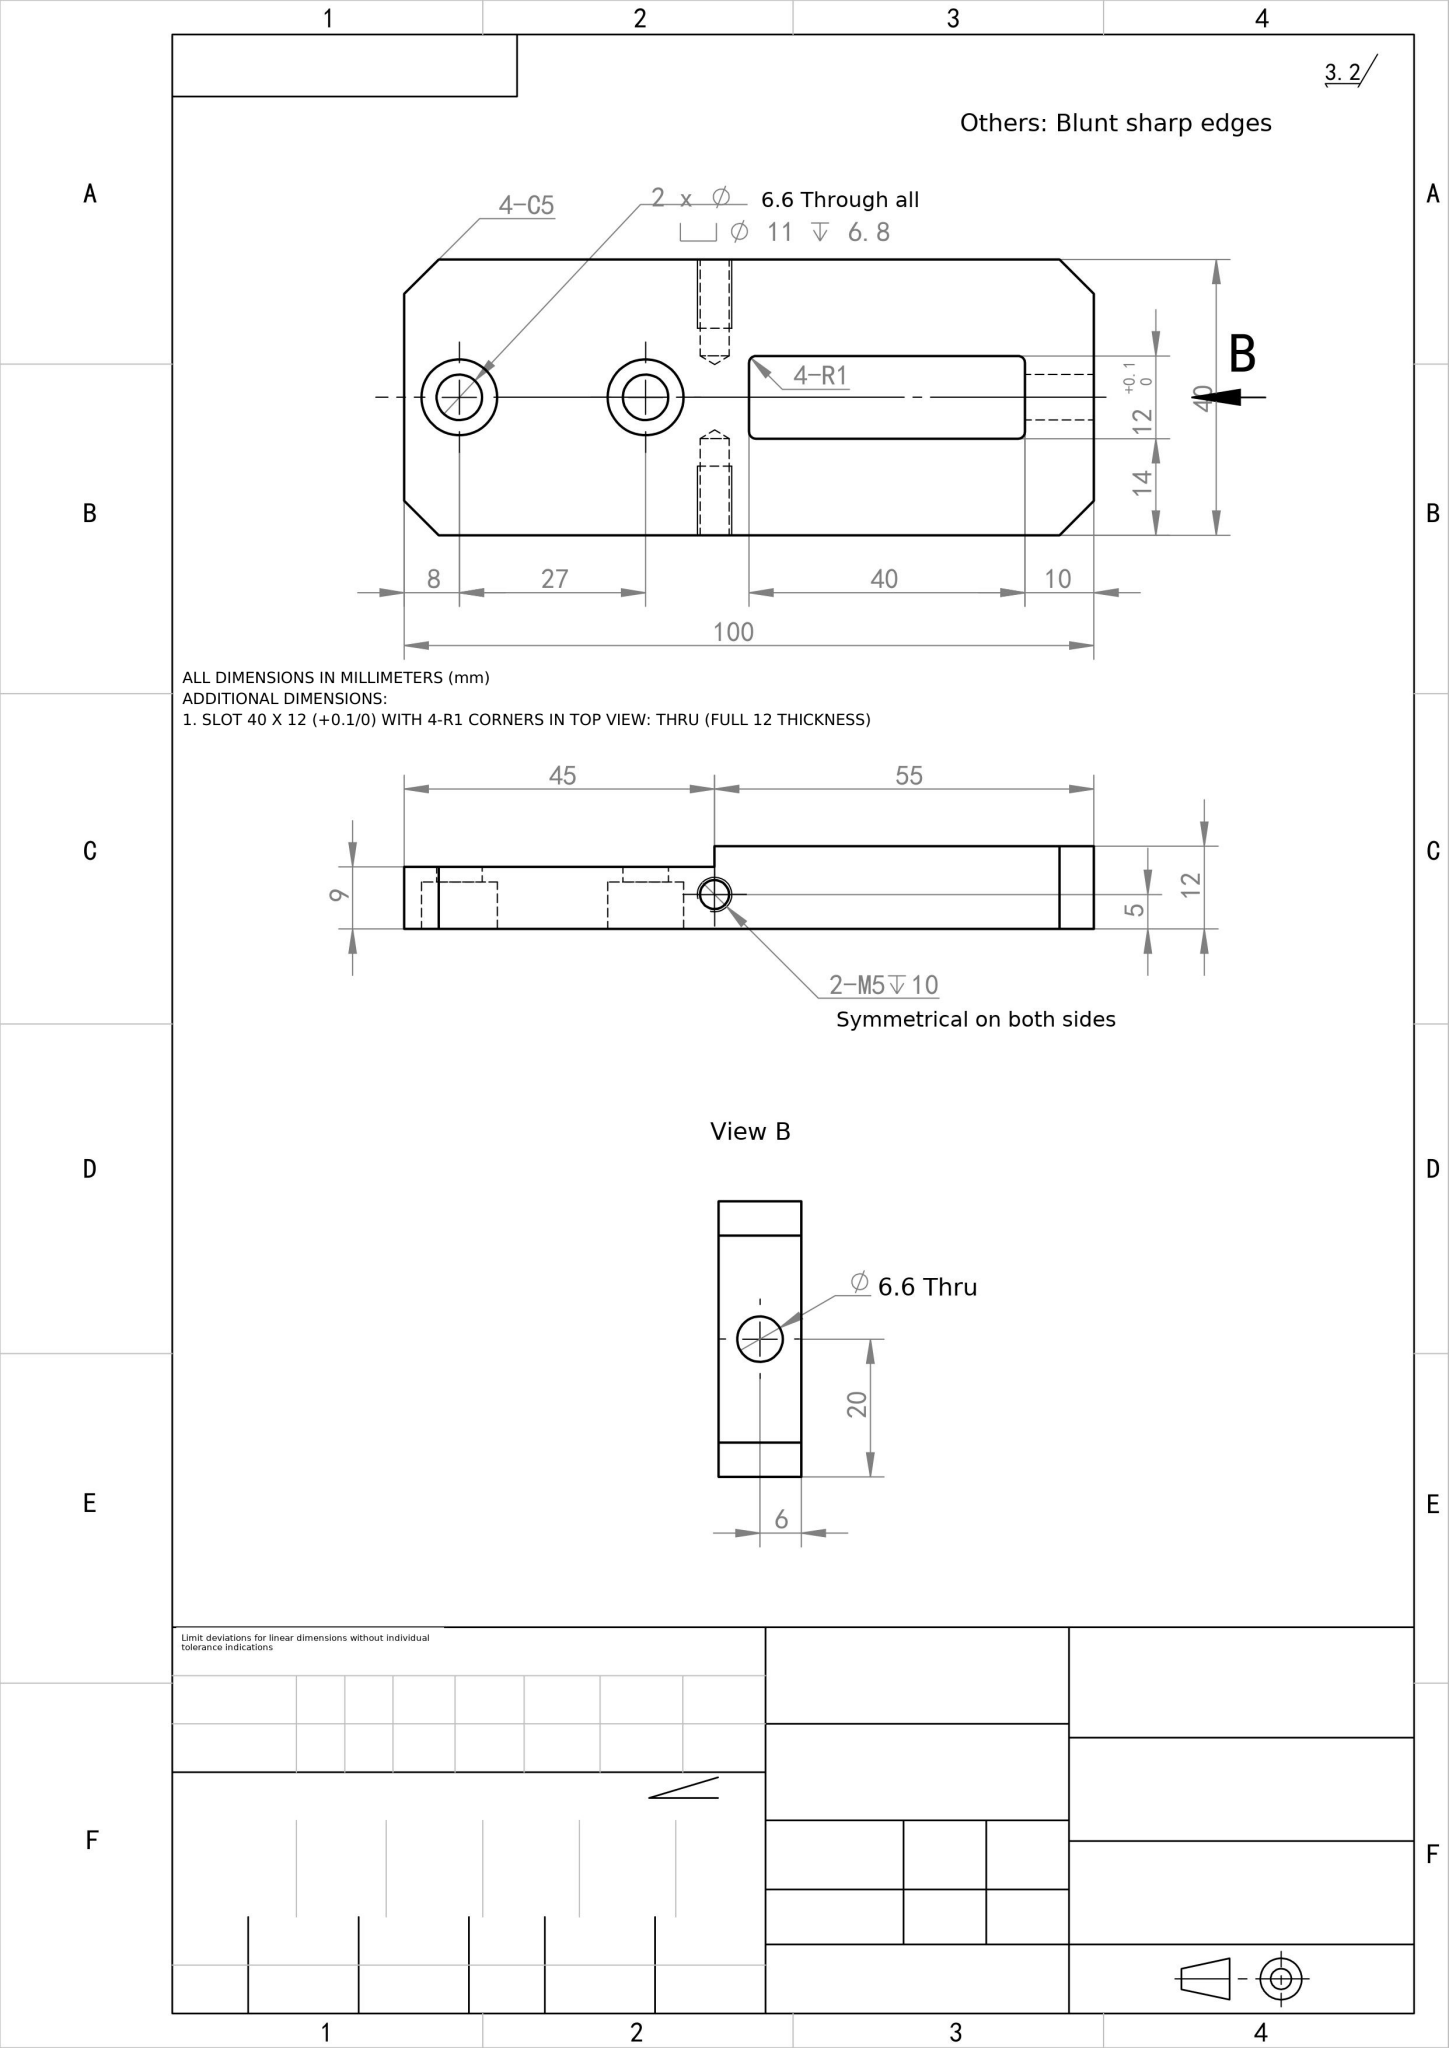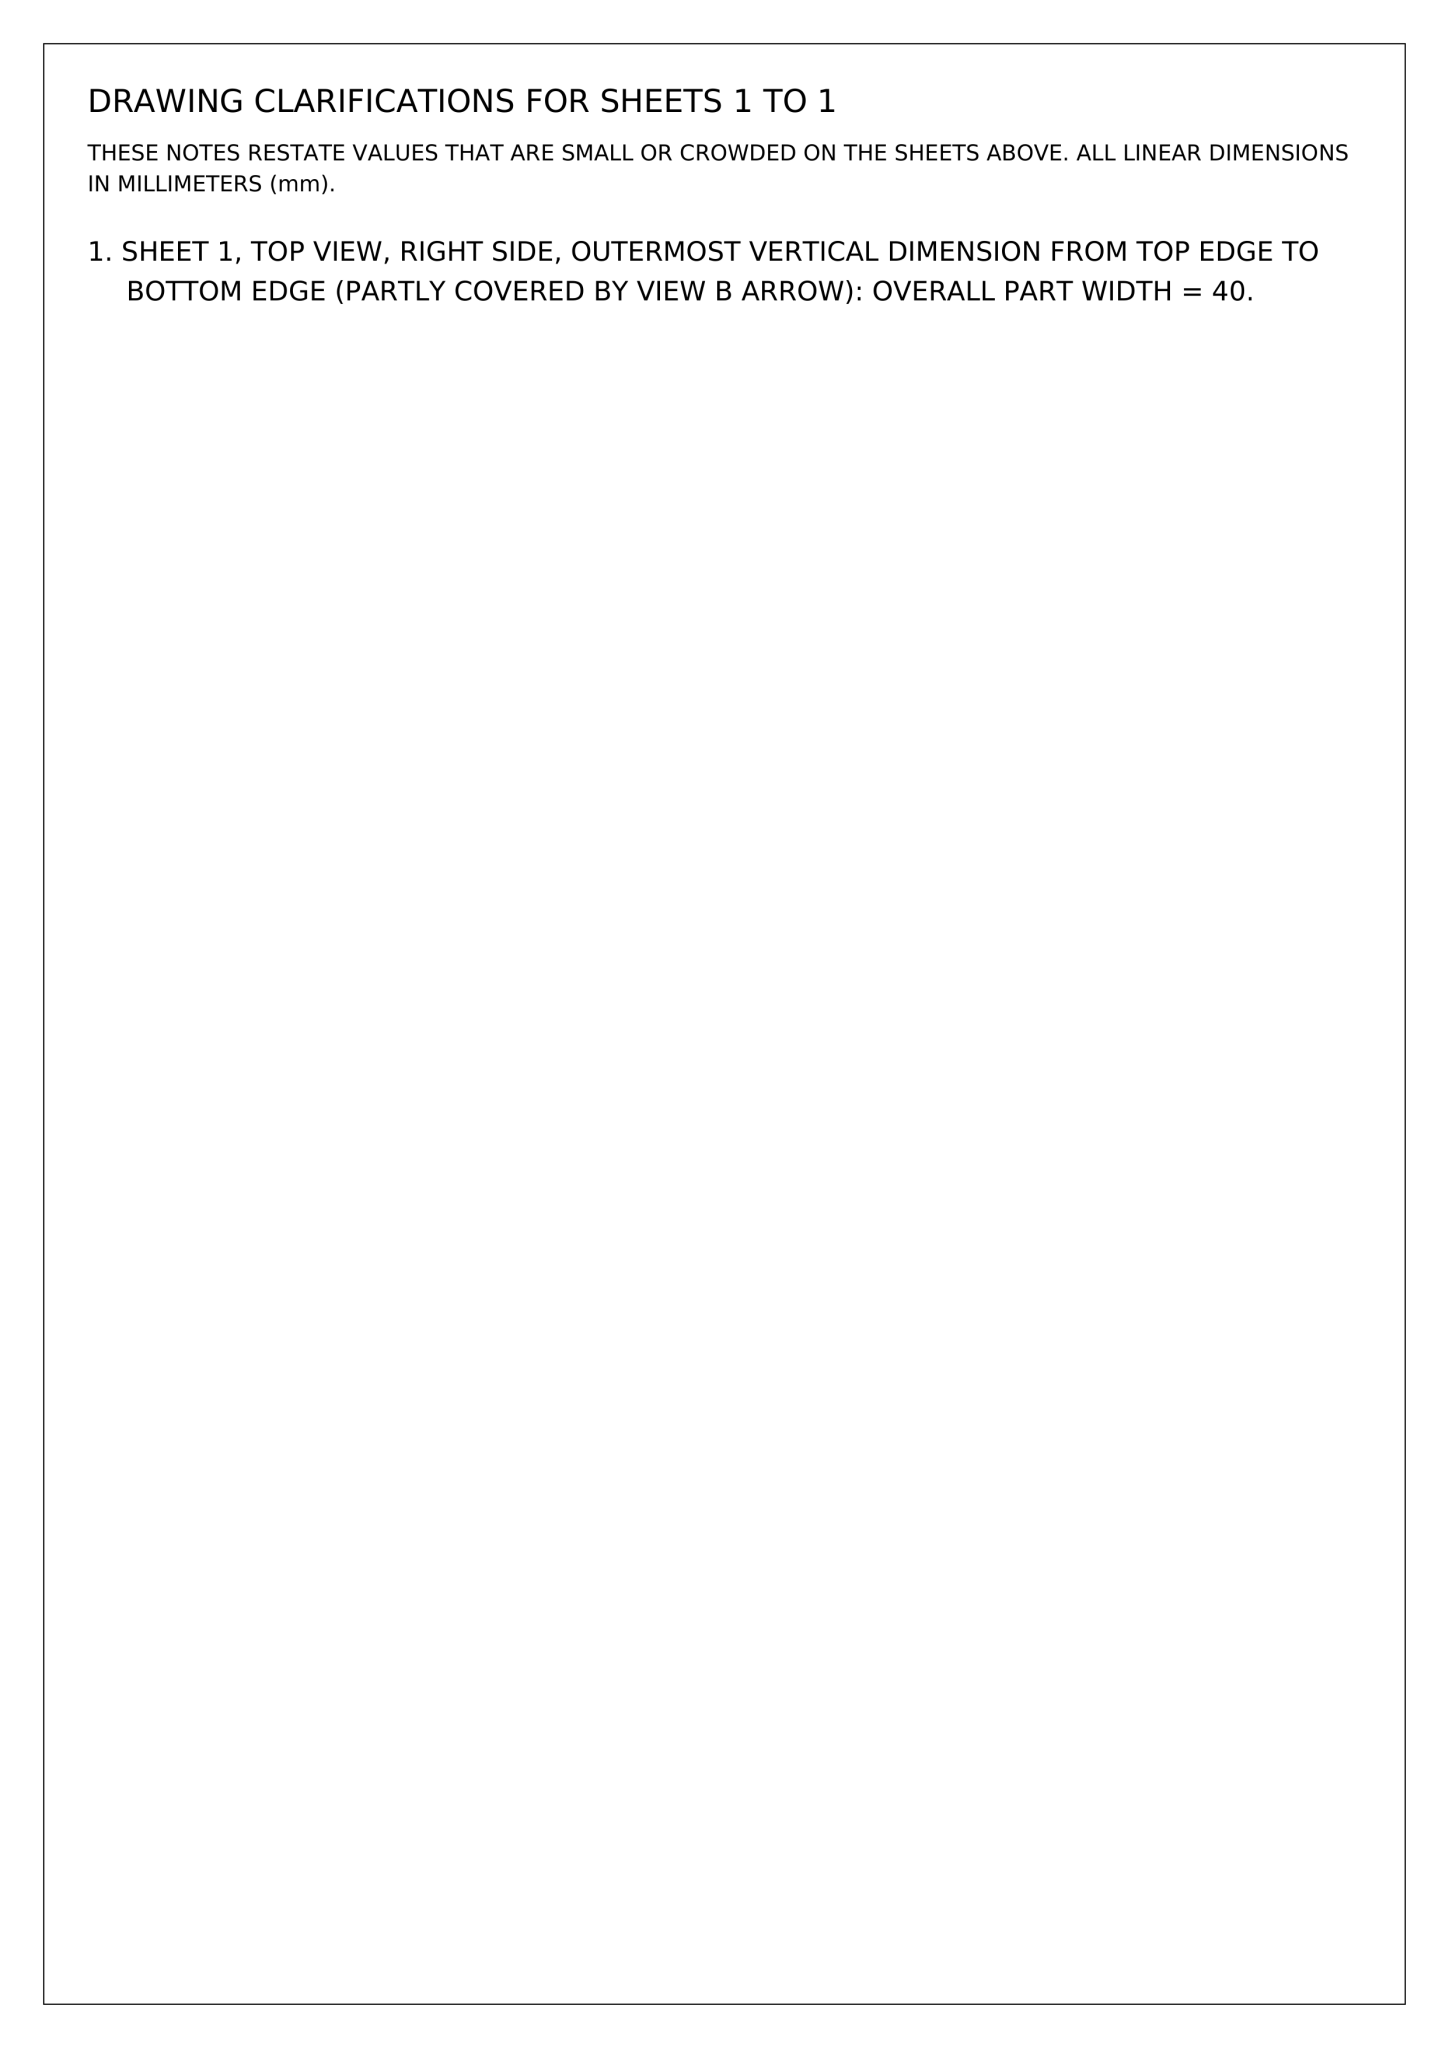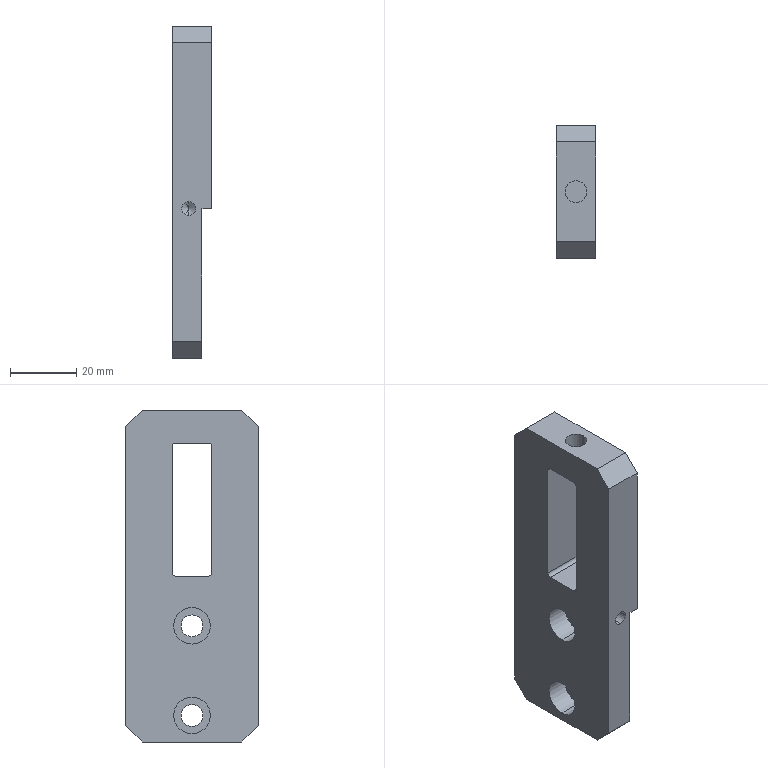Part | NX | mm | 1 solid | 40 faces | box 12 x 40 x 100 mm | volume 34141 mm3 | cylinder 18 | plane 18 | cone 4 | commonest cylinder face diameters 6.6 x6 4.2 x4 11 x4 2 x4